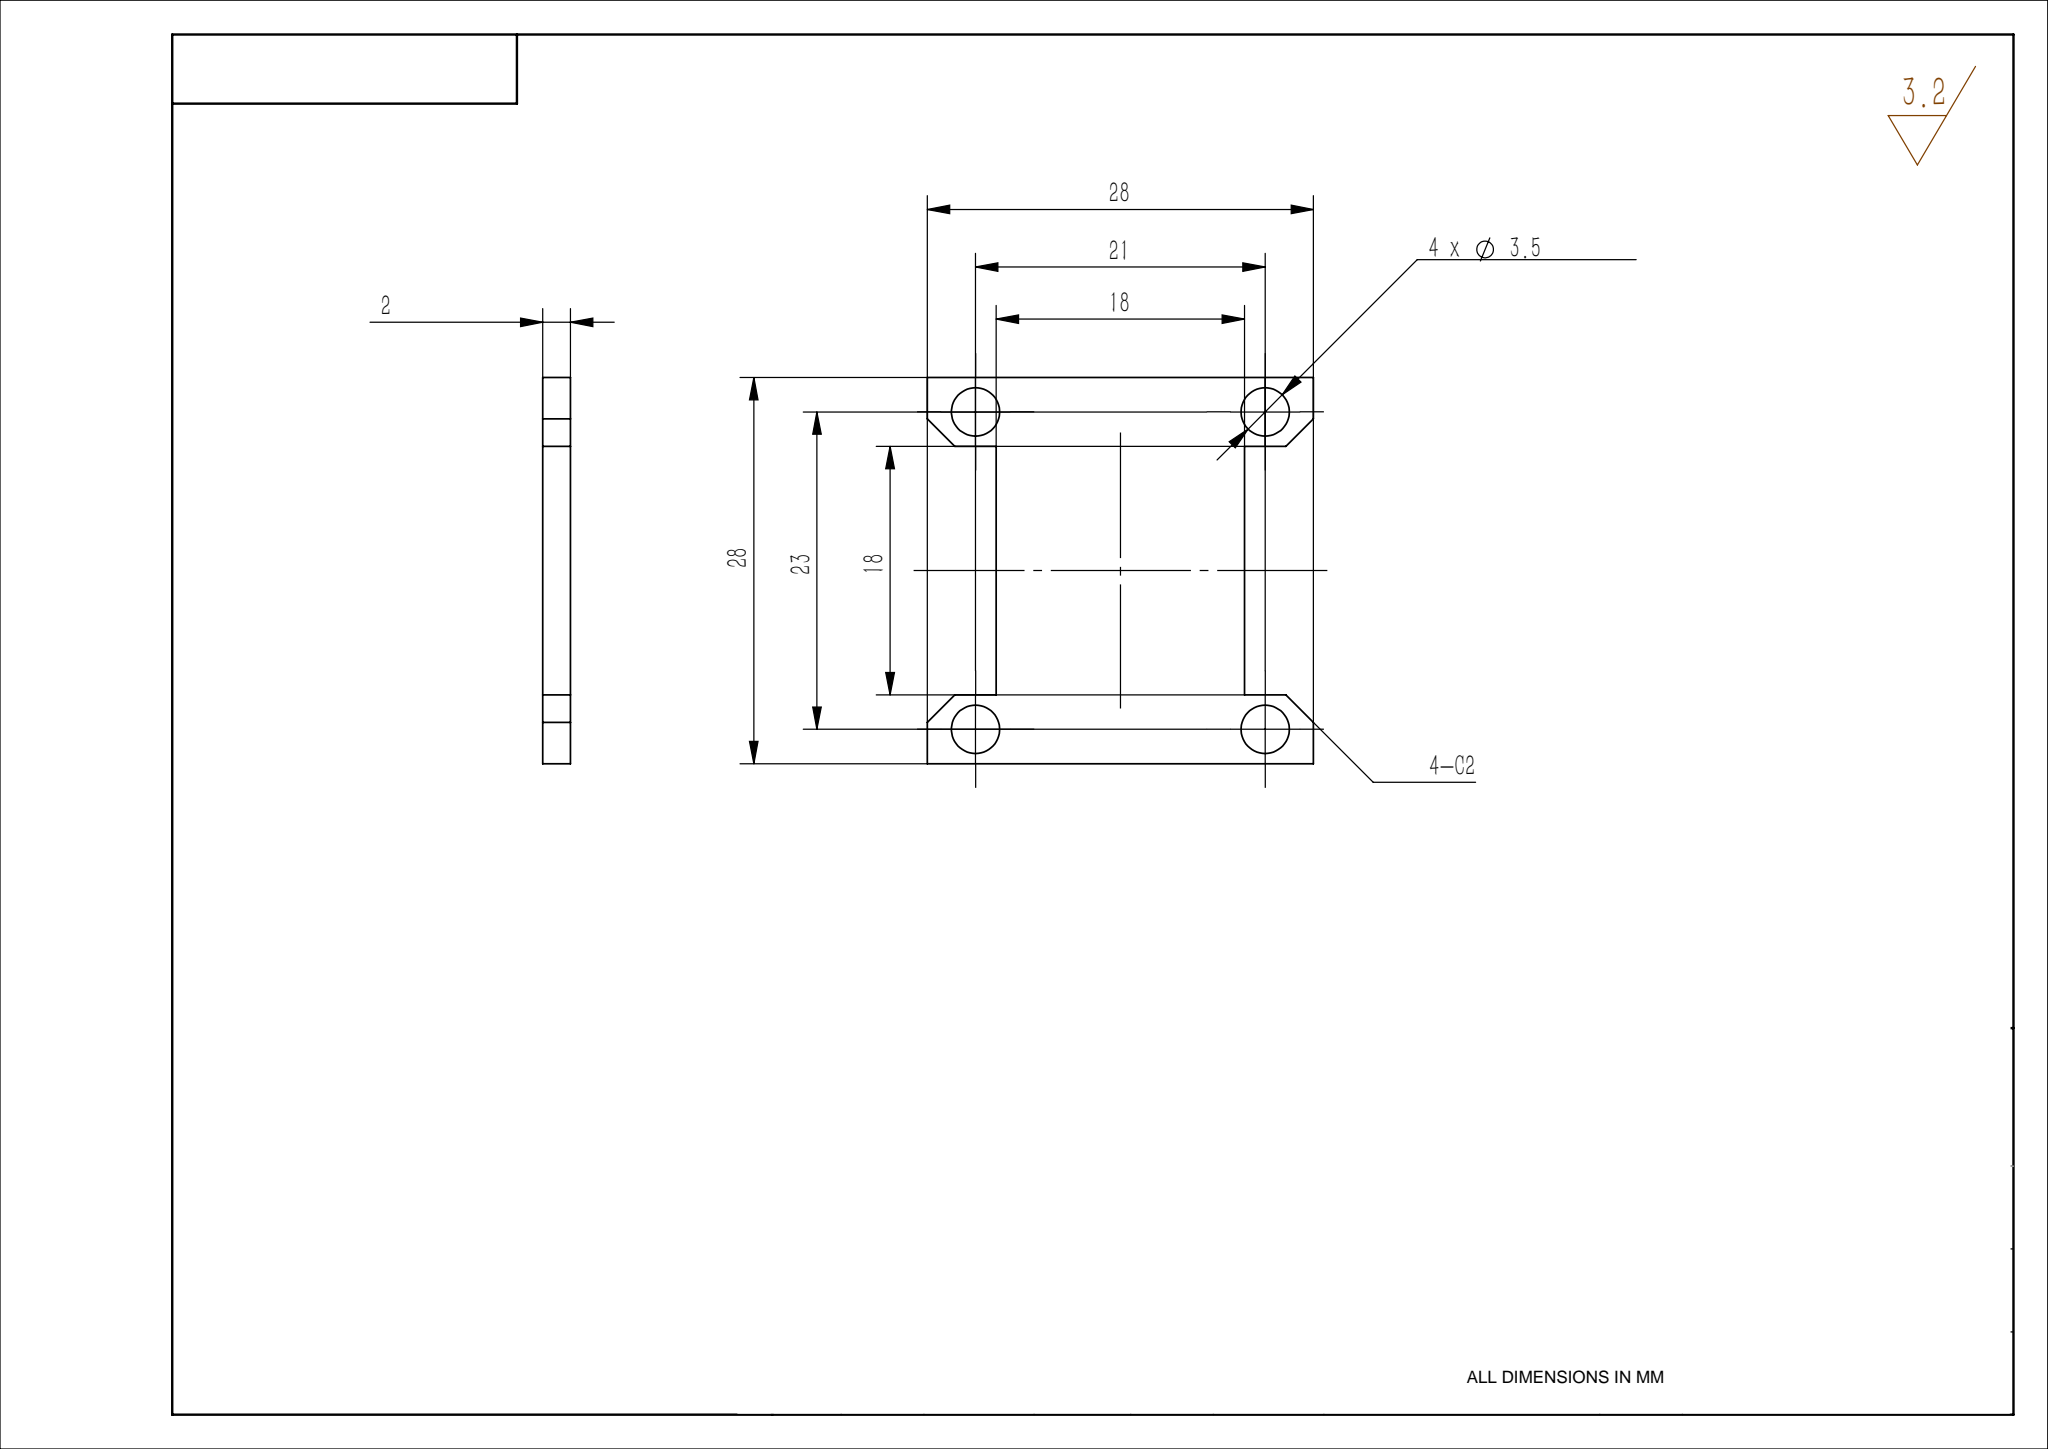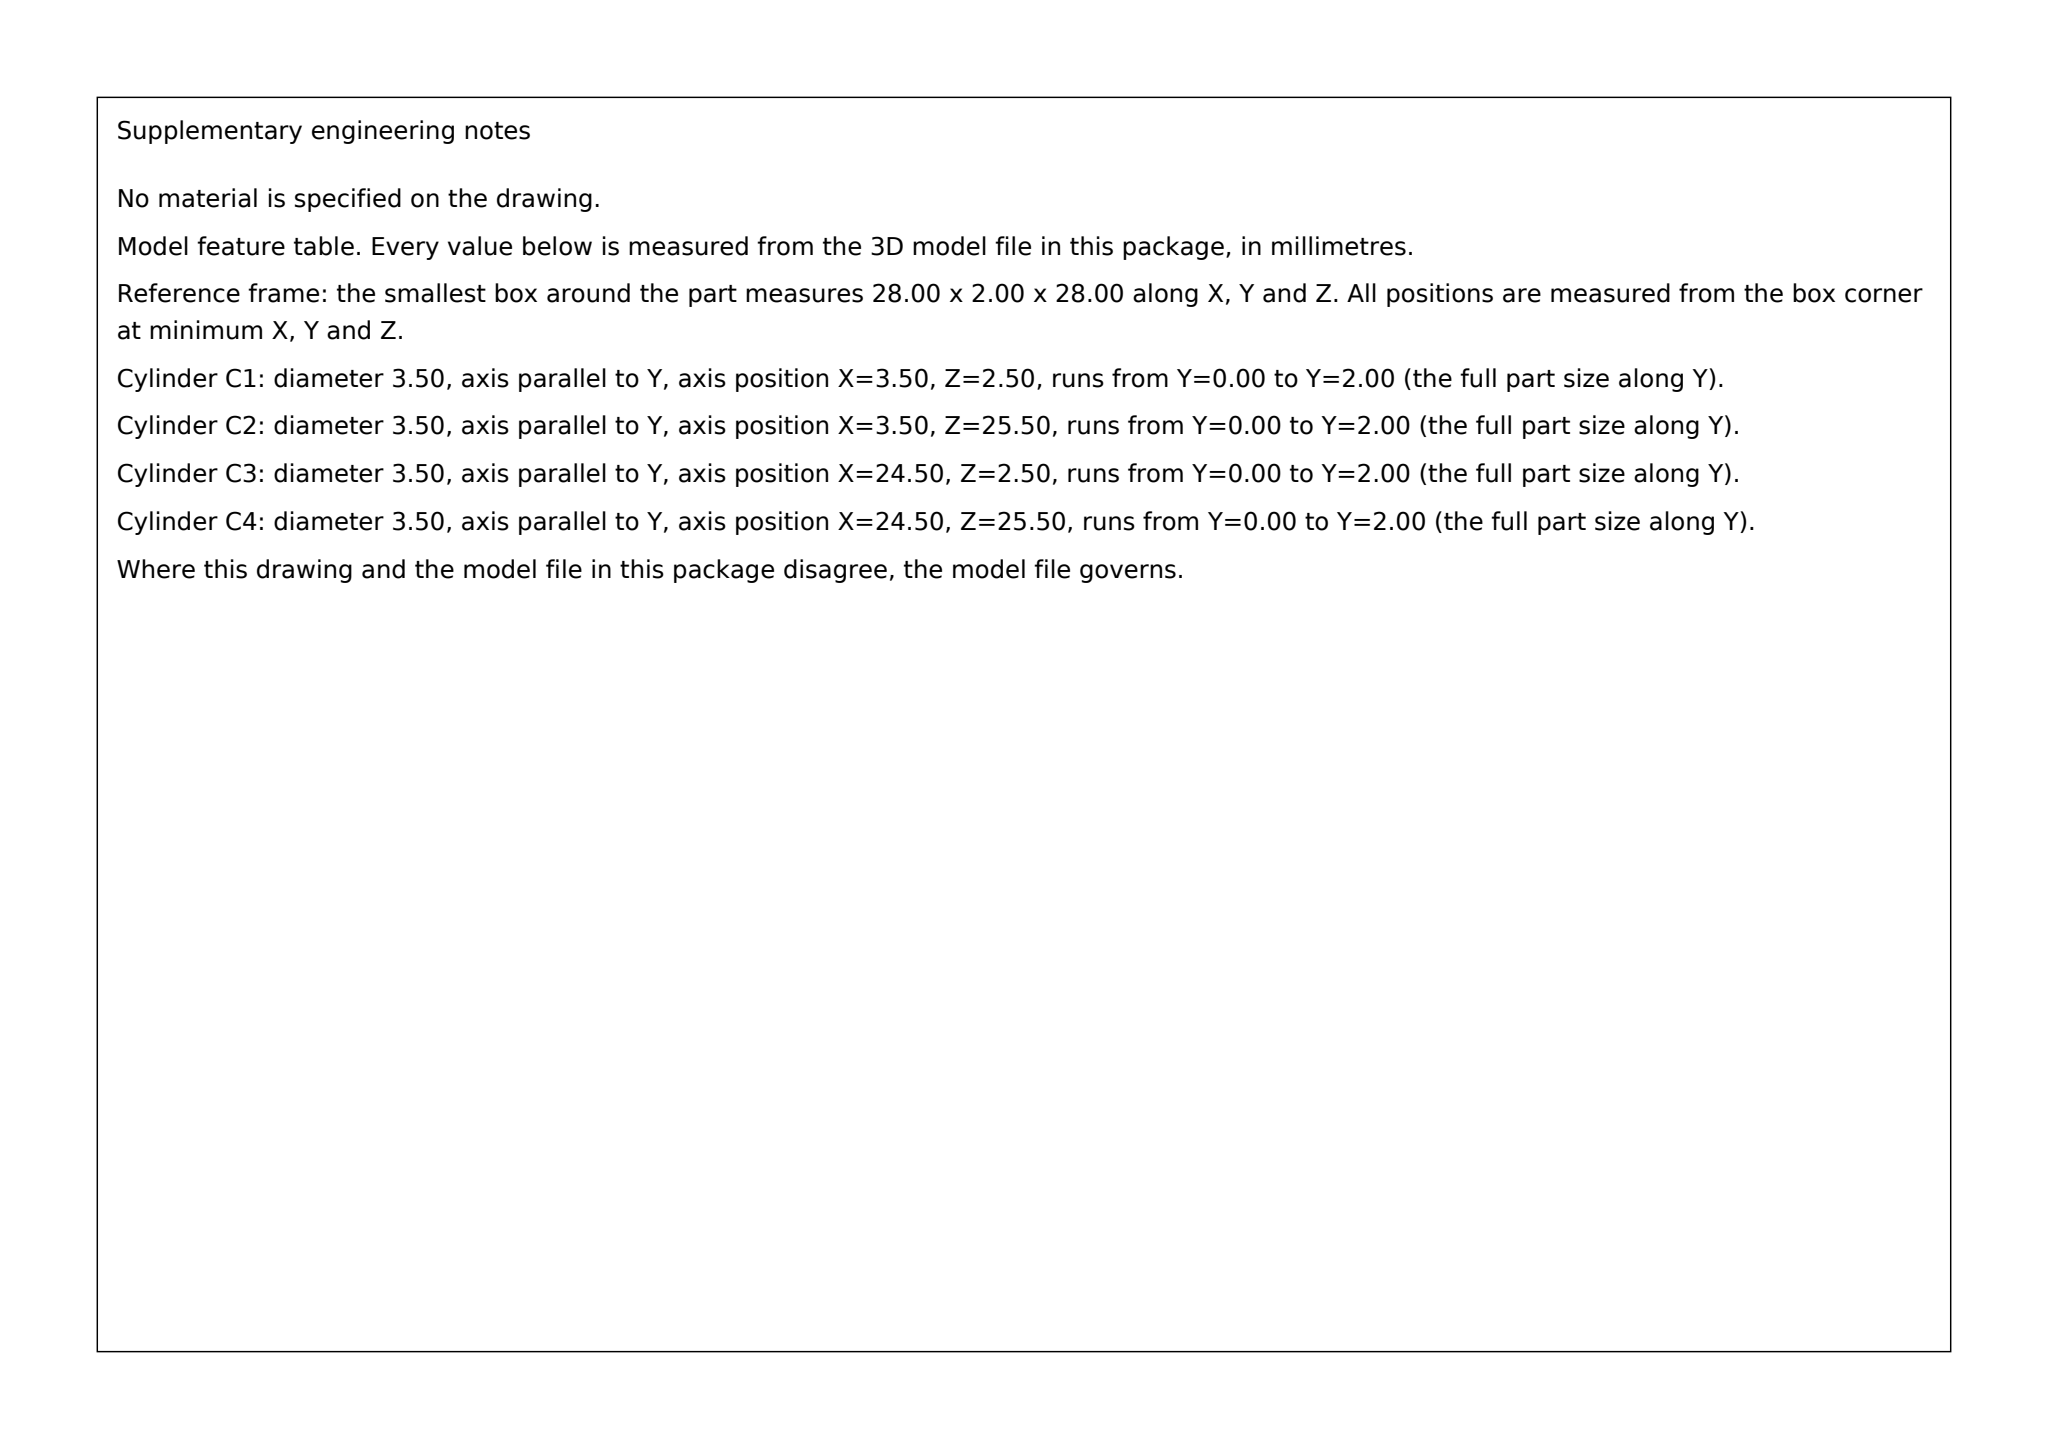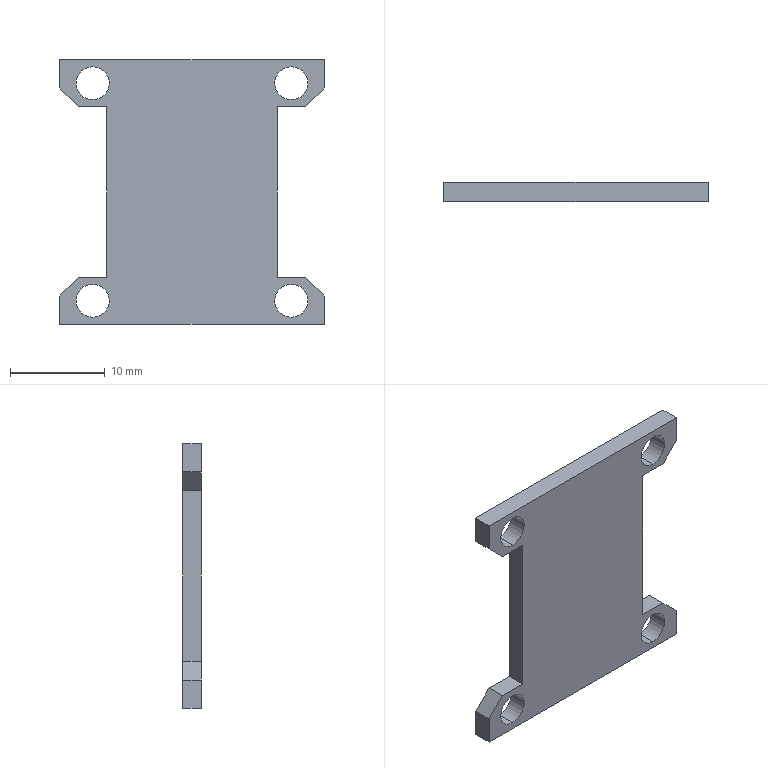Part | SolidWorks | mm | 1 solid | 26 faces | box 28 x 2 x 28 mm | volume 1115 mm3 | plane 18 | cylinder 8 | commonest cylinder face diameters 3.5 x8
STEP:
#1=CARTESIAN_POINT('',(-10.5,-2.,-13.25));
#2=VERTEX_POINT('',#1);
#3=CARTESIAN_POINT('',(-10.5,-2.,-9.75));
#4=VERTEX_POINT('',#3);
#5=CARTESIAN_POINT('',(-10.5,-2.,-11.5));
#6=DIRECTION('',(0.,1.,0.));
#7=DIRECTION('',(0.,0.,1.));
#8=AXIS2_PLACEMENT_3D('',#5,#6,#7);
#9=CIRCLE('',#8,1.75);
#10=EDGE_CURVE('',#2,#4,#9,.T.);
#11=ORIENTED_EDGE('',*,*,#10,.F.);
#12=CARTESIAN_POINT('',(-10.5,0.,-13.25));
#13=VERTEX_POINT('',#12);
#14=CARTESIAN_POINT('',(-10.5,0.,-13.25));
#15=DIRECTION('',(0.,1.,0.));
#16=VECTOR('',#15,1000.);
#17=LINE('',#14,#16);
#18=EDGE_CURVE('',#2,#13,#17,.T.);
#19=ORIENTED_EDGE('',*,*,#18,.T.);
#20=CARTESIAN_POINT('',(-10.5,0.,-9.75));
#21=VERTEX_POINT('',#20);
#22=CARTESIAN_POINT('',(-10.5,0.,-11.5));
#23=DIRECTION('',(0.,1.,0.));
#24=DIRECTION('',(0.,0.,1.));
#25=AXIS2_PLACEMENT_3D('',#22,#23,#24);
#26=CIRCLE('',#25,1.75);
#27=EDGE_CURVE('',#13,#21,#26,.T.);
#28=ORIENTED_EDGE('',*,*,#27,.T.);
#29=CARTESIAN_POINT('',(-10.5,0.,-9.75));
#30=DIRECTION('',(0.,1.,0.));
#31=VECTOR('',#30,1000.);
#32=LINE('',#29,#31);
#33=EDGE_CURVE('',#4,#21,#32,.T.);
#34=ORIENTED_EDGE('',*,*,#33,.F.);
#35=EDGE_LOOP('',(#11,#19,#28,#34));
#36=FACE_OUTER_BOUND('',#35,.T.);
#37=CARTESIAN_POINT('',(-10.5,0.,-11.5));
#38=DIRECTION('',(0.,1.,0.));
#39=DIRECTION('',(0.,0.,1.));
#40=AXIS2_PLACEMENT_3D('',#37,#38,#39);
#41=CYLINDRICAL_SURFACE('',#40,1.75);
#42=ADVANCED_FACE('',(#36),#41,.F.);
#43=CARTESIAN_POINT('',(10.5,-2.,-13.25));
#44=VERTEX_POINT('',#43);
#45=CARTESIAN_POINT('',(10.5,-2.,-9.75));
#46=VERTEX_POINT('',#45);
#47=CARTESIAN_POINT('',(10.5,-2.,-11.5));
#48=DIRECTION('',(0.,1.,0.));
#49=DIRECTION('',(0.,0.,1.));
#50=AXIS2_PLACEMENT_3D('',#47,#48,#49);
#51=CIRCLE('',#50,1.75);
#52=EDGE_CURVE('',#44,#46,#51,.T.);
#53=ORIENTED_EDGE('',*,*,#52,.F.);
#54=CARTESIAN_POINT('',(10.5,0.,-13.25));
#55=VERTEX_POINT('',#54);
#56=CARTESIAN_POINT('',(10.5,0.,-13.25));
#57=DIRECTION('',(0.,1.,0.));
#58=VECTOR('',#57,1000.);
#59=LINE('',#56,#58);
#60=EDGE_CURVE('',#44,#55,#59,.T.);
#61=ORIENTED_EDGE('',*,*,#60,.T.);
#62=CARTESIAN_POINT('',(10.5,0.,-9.75));
#63=VERTEX_POINT('',#62);
#64=CARTESIAN_POINT('',(10.5,0.,-11.5));
#65=DIRECTION('',(0.,1.,0.));
#66=DIRECTION('',(0.,0.,1.));
#67=AXIS2_PLACEMENT_3D('',#64,#65,#66);
#68=CIRCLE('',#67,1.75);
#69=EDGE_CURVE('',#55,#63,#68,.T.);
#70=ORIENTED_EDGE('',*,*,#69,.T.);
#71=CARTESIAN_POINT('',(10.5,0.,-9.75));
#72=DIRECTION('',(0.,1.,0.));
#73=VECTOR('',#72,1000.);
#74=LINE('',#71,#73);
#75=EDGE_CURVE('',#46,#63,#74,.T.);
#76=ORIENTED_EDGE('',*,*,#75,.F.);
#77=EDGE_LOOP('',(#53,#61,#70,#76));
#78=FACE_OUTER_BOUND('',#77,.T.);
#79=CARTESIAN_POINT('',(10.5,0.,-11.5));
#80=DIRECTION('',(0.,1.,0.));
#81=DIRECTION('',(0.,0.,1.));
#82=AXIS2_PLACEMENT_3D('',#79,#80,#81);
#83=CYLINDRICAL_SURFACE('',#82,1.75);
#84=ADVANCED_FACE('',(#78),#83,.F.);
#85=CARTESIAN_POINT('',(10.5,-2.,9.75));
#86=VERTEX_POINT('',#85);
#87=CARTESIAN_POINT('',(10.5,-2.,13.25));
#88=VERTEX_POINT('',#87);
#89=CARTESIAN_POINT('',(10.5,-2.,11.5));
#90=DIRECTION('',(0.,1.,0.));
#91=DIRECTION('',(0.,0.,1.));
#92=AXIS2_PLACEMENT_3D('',#89,#90,#91);
#93=CIRCLE('',#92,1.75);
#94=EDGE_CURVE('',#86,#88,#93,.T.);
#95=ORIENTED_EDGE('',*,*,#94,.F.);
#96=CARTESIAN_POINT('',(10.5,0.,9.75));
#97=VERTEX_POINT('',#96);
#98=CARTESIAN_POINT('',(10.5,0.,9.75));
#99=DIRECTION('',(0.,1.,0.));
#100=VECTOR('',#99,1000.);
#101=LINE('',#98,#100);
#102=EDGE_CURVE('',#86,#97,#101,.T.);
#103=ORIENTED_EDGE('',*,*,#102,.T.);
#104=CARTESIAN_POINT('',(10.5,0.,13.25));
#105=VERTEX_POINT('',#104);
#106=CARTESIAN_POINT('',(10.5,0.,11.5));
#107=DIRECTION('',(0.,1.,0.));
#108=DIRECTION('',(0.,0.,1.));
#109=AXIS2_PLACEMENT_3D('',#106,#107,#108);
#110=CIRCLE('',#109,1.75);
#111=EDGE_CURVE('',#97,#105,#110,.T.);
#112=ORIENTED_EDGE('',*,*,#111,.T.);
#113=CARTESIAN_POINT('',(10.5,0.,13.25));
#114=DIRECTION('',(0.,1.,0.));
#115=VECTOR('',#114,1000.);
#116=LINE('',#113,#115);
#117=EDGE_CURVE('',#88,#105,#116,.T.);
#118=ORIENTED_EDGE('',*,*,#117,.F.);
#119=EDGE_LOOP('',(#95,#103,#112,#118));
#120=FACE_OUTER_BOUND('',#119,.T.);
#121=CARTESIAN_POINT('',(10.5,0.,11.5));
#122=DIRECTION('',(0.,1.,0.));
#123=DIRECTION('',(0.,0.,1.));
#124=AXIS2_PLACEMENT_3D('',#121,#122,#123);
#125=CYLINDRICAL_SURFACE('',#124,1.75);
#126=ADVANCED_FACE('',(#120),#125,.F.);
#127=CARTESIAN_POINT('',(-10.5,-2.,9.75));
#128=VERTEX_POINT('',#127);
#129=CARTESIAN_POINT('',(-10.5,-2.,13.25));
#130=VERTEX_POINT('',#129);
#131=CARTESIAN_POINT('',(-10.5,-2.,11.5));
#132=DIRECTION('',(0.,1.,0.));
#133=DIRECTION('',(0.,0.,1.));
#134=AXIS2_PLACEMENT_3D('',#131,#132,#133);
#135=CIRCLE('',#134,1.75);
#136=EDGE_CURVE('',#128,#130,#135,.T.);
#137=ORIENTED_EDGE('',*,*,#136,.F.);
#138=CARTESIAN_POINT('',(-10.5,0.,9.75));
#139=VERTEX_POINT('',#138);
#140=CARTESIAN_POINT('',(-10.5,0.,9.75));
#141=DIRECTION('',(0.,1.,0.));
#142=VECTOR('',#141,1000.);
#143=LINE('',#140,#142);
#144=EDGE_CURVE('',#128,#139,#143,.T.);
#145=ORIENTED_EDGE('',*,*,#144,.T.);
#146=CARTESIAN_POINT('',(-10.5,0.,13.25));
#147=VERTEX_POINT('',#146);
#148=CARTESIAN_POINT('',(-10.5,0.,11.5));
#149=DIRECTION('',(0.,1.,0.));
#150=DIRECTION('',(0.,0.,1.));
#151=AXIS2_PLACEMENT_3D('',#148,#149,#150);
#152=CIRCLE('',#151,1.75);
#153=EDGE_CURVE('',#139,#147,#152,.T.);
#154=ORIENTED_EDGE('',*,*,#153,.T.);
#155=CARTESIAN_POINT('',(-10.5,0.,13.25));
#156=DIRECTION('',(0.,1.,0.));
#157=VECTOR('',#156,1000.);
#158=LINE('',#155,#157);
#159=EDGE_CURVE('',#130,#147,#158,.T.);
#160=ORIENTED_EDGE('',*,*,#159,.F.);
#161=EDGE_LOOP('',(#137,#145,#154,#160));
#162=FACE_OUTER_BOUND('',#161,.T.);
#163=CARTESIAN_POINT('',(-10.5,0.,11.5));
#164=DIRECTION('',(0.,1.,0.));
#165=DIRECTION('',(0.,0.,1.));
#166=AXIS2_PLACEMENT_3D('',#163,#164,#165);
#167=CYLINDRICAL_SURFACE('',#166,1.75);
#168=ADVANCED_FACE('',(#162),#167,.F.);
#169=CARTESIAN_POINT('',(14.,0.,-11.));
#170=VERTEX_POINT('',#169);
#171=CARTESIAN_POINT('',(14.,0.,-14.));
#172=VERTEX_POINT('',#171);
#173=CARTESIAN_POINT('',(14.,0.,14.));
#174=DIRECTION('',(0.,0.,-1.));
#175=VECTOR('',#174,1000.);
#176=LINE('',#173,#175);
#177=EDGE_CURVE('',#170,#172,#176,.T.);
#178=ORIENTED_EDGE('',*,*,#177,.F.);
#179=CARTESIAN_POINT('',(14.,-2.,-11.));
#180=VERTEX_POINT('',#179);
#181=CARTESIAN_POINT('',(14.,-2.,-11.));
#182=DIRECTION('',(0.,-1.,0.));
#183=VECTOR('',#182,1000.);
#184=LINE('',#181,#183);
#185=EDGE_CURVE('',#170,#180,#184,.T.);
#186=ORIENTED_EDGE('',*,*,#185,.T.);
#187=CARTESIAN_POINT('',(14.,-2.,-14.));
#188=VERTEX_POINT('',#187);
#189=CARTESIAN_POINT('',(14.,-2.,14.));
#190=DIRECTION('',(0.,0.,-1.));
#191=VECTOR('',#190,1000.);
#192=LINE('',#189,#191);
#193=EDGE_CURVE('',#180,#188,#192,.T.);
#194=ORIENTED_EDGE('',*,*,#193,.T.);
#195=CARTESIAN_POINT('',(14.,-2.,-14.));
#196=DIRECTION('',(0.,1.,0.));
#197=VECTOR('',#196,1000.);
#198=LINE('',#195,#197);
#199=EDGE_CURVE('',#188,#172,#198,.T.);
#200=ORIENTED_EDGE('',*,*,#199,.T.);
#201=EDGE_LOOP('',(#178,#186,#194,#200));
#202=FACE_OUTER_BOUND('',#201,.T.);
#203=CARTESIAN_POINT('',(14.,-2.,14.));
#204=DIRECTION('',(1.,0.,0.));
#205=DIRECTION('',(0.,0.,-1.));
#206=AXIS2_PLACEMENT_3D('',#203,#204,#205);
#207=PLANE('',#206);
#208=ADVANCED_FACE('',(#202),#207,.T.);
#209=CARTESIAN_POINT('',(-14.,-2.,-14.));
#210=VERTEX_POINT('',#209);
#211=CARTESIAN_POINT('',(-14.,-2.,-11.));
#212=VERTEX_POINT('',#211);
#213=CARTESIAN_POINT('',(-14.,-2.,14.));
#214=DIRECTION('',(0.,0.,1.));
#215=VECTOR('',#214,1000.);
#216=LINE('',#213,#215);
#217=EDGE_CURVE('',#210,#212,#216,.T.);
#218=ORIENTED_EDGE('',*,*,#217,.T.);
#219=CARTESIAN_POINT('',(-14.,0.,-11.));
#220=VERTEX_POINT('',#219);
#221=CARTESIAN_POINT('',(-14.,0.,-11.));
#222=DIRECTION('',(0.,1.,0.));
#223=VECTOR('',#222,1000.);
#224=LINE('',#221,#223);
#225=EDGE_CURVE('',#212,#220,#224,.T.);
#226=ORIENTED_EDGE('',*,*,#225,.T.);
#227=CARTESIAN_POINT('',(-14.,0.,-14.));
#228=VERTEX_POINT('',#227);
#229=CARTESIAN_POINT('',(-14.,0.,14.));
#230=DIRECTION('',(0.,0.,1.));
#231=VECTOR('',#230,1000.);
#232=LINE('',#229,#231);
#233=EDGE_CURVE('',#228,#220,#232,.T.);
#234=ORIENTED_EDGE('',*,*,#233,.F.);
#235=CARTESIAN_POINT('',(-14.,-2.,-14.));
#236=DIRECTION('',(0.,1.,0.));
#237=VECTOR('',#236,1000.);
#238=LINE('',#235,#237);
#239=EDGE_CURVE('',#210,#228,#238,.T.);
#240=ORIENTED_EDGE('',*,*,#239,.F.);
#241=EDGE_LOOP('',(#218,#226,#234,#240));
#242=FACE_OUTER_BOUND('',#241,.T.);
#243=CARTESIAN_POINT('',(-14.,-2.,14.));
#244=DIRECTION('',(-1.,0.,0.));
#245=DIRECTION('',(0.,0.,1.));
#246=AXIS2_PLACEMENT_3D('',#243,#244,#245);
#247=PLANE('',#246);
#248=ADVANCED_FACE('',(#242),#247,.T.);
#249=CARTESIAN_POINT('',(14.,-2.,14.));
#250=VERTEX_POINT('',#249);
#251=CARTESIAN_POINT('',(14.,-2.,11.));
#252=VERTEX_POINT('',#251);
#253=CARTESIAN_POINT('',(14.,-2.,14.));
#254=DIRECTION('',(0.,0.,-1.));
#255=VECTOR('',#254,1000.);
#256=LINE('',#253,#255);
#257=EDGE_CURVE('',#250,#252,#256,.T.);
#258=ORIENTED_EDGE('',*,*,#257,.T.);
#259=CARTESIAN_POINT('',(14.,0.,11.));
#260=VERTEX_POINT('',#259);
#261=CARTESIAN_POINT('',(14.,0.,11.));
#262=DIRECTION('',(0.,1.,0.));
#263=VECTOR('',#262,1000.);
#264=LINE('',#261,#263);
#265=EDGE_CURVE('',#252,#260,#264,.T.);
#266=ORIENTED_EDGE('',*,*,#265,.T.);
#267=CARTESIAN_POINT('',(14.,0.,14.));
#268=VERTEX_POINT('',#267);
#269=CARTESIAN_POINT('',(14.,0.,14.));
#270=DIRECTION('',(0.,0.,-1.));
#271=VECTOR('',#270,1000.);
#272=LINE('',#269,#271);
#273=EDGE_CURVE('',#268,#260,#272,.T.);
#274=ORIENTED_EDGE('',*,*,#273,.F.);
#275=CARTESIAN_POINT('',(14.,-2.,14.));
#276=DIRECTION('',(0.,1.,0.));
#277=VECTOR('',#276,1000.);
#278=LINE('',#275,#277);
#279=EDGE_CURVE('',#250,#268,#278,.T.);
#280=ORIENTED_EDGE('',*,*,#279,.F.);
#281=EDGE_LOOP('',(#258,#266,#274,#280));
#282=FACE_OUTER_BOUND('',#281,.T.);
#283=CARTESIAN_POINT('',(14.,-2.,14.));
#284=DIRECTION('',(1.,0.,0.));
#285=DIRECTION('',(0.,0.,-1.));
#286=AXIS2_PLACEMENT_3D('',#283,#284,#285);
#287=PLANE('',#286);
#288=ADVANCED_FACE('',(#282),#287,.T.);
#289=CARTESIAN_POINT('',(-14.,0.,14.));
#290=VERTEX_POINT('',#289);
#291=CARTESIAN_POINT('',(-14.,0.,14.));
#292=DIRECTION('',(1.,0.,0.));
#293=VECTOR('',#292,1000.);
#294=LINE('',#291,#293);
#295=EDGE_CURVE('',#290,#268,#294,.T.);
#296=ORIENTED_EDGE('',*,*,#295,.F.);
#297=CARTESIAN_POINT('',(-14.,-2.,14.));
#298=VERTEX_POINT('',#297);
#299=CARTESIAN_POINT('',(-14.,-2.,14.));
#300=DIRECTION('',(0.,1.,0.));
#301=VECTOR('',#300,1000.);
#302=LINE('',#299,#301);
#303=EDGE_CURVE('',#298,#290,#302,.T.);
#304=ORIENTED_EDGE('',*,*,#303,.F.);
#305=CARTESIAN_POINT('',(-14.,-2.,14.));
#306=DIRECTION('',(1.,0.,0.));
#307=VECTOR('',#306,1000.);
#308=LINE('',#305,#307);
#309=EDGE_CURVE('',#298,#250,#308,.T.);
#310=ORIENTED_EDGE('',*,*,#309,.T.);
#311=ORIENTED_EDGE('',*,*,#279,.T.);
#312=EDGE_LOOP('',(#296,#304,#310,#311));
#313=FACE_OUTER_BOUND('',#312,.T.);
#314=CARTESIAN_POINT('',(-14.,-2.,14.));
#315=DIRECTION('',(0.,0.,1.));
#316=DIRECTION('',(1.,0.,0.));
#317=AXIS2_PLACEMENT_3D('',#314,#315,#316);
#318=PLANE('',#317);
#319=ADVANCED_FACE('',(#313),#318,.T.);
#320=CARTESIAN_POINT('',(-14.,0.,11.));
#321=VERTEX_POINT('',#320);
#322=CARTESIAN_POINT('',(-14.,0.,14.));
#323=DIRECTION('',(0.,0.,1.));
#324=VECTOR('',#323,1000.);
#325=LINE('',#322,#324);
#326=EDGE_CURVE('',#321,#290,#325,.T.);
#327=ORIENTED_EDGE('',*,*,#326,.F.);
#328=CARTESIAN_POINT('',(-14.,-2.,11.));
#329=VERTEX_POINT('',#328);
#330=CARTESIAN_POINT('',(-14.,-2.,11.));
#331=DIRECTION('',(0.,-1.,0.));
#332=VECTOR('',#331,1000.);
#333=LINE('',#330,#332);
#334=EDGE_CURVE('',#321,#329,#333,.T.);
#335=ORIENTED_EDGE('',*,*,#334,.T.);
#336=CARTESIAN_POINT('',(-14.,-2.,14.));
#337=DIRECTION('',(0.,0.,1.));
#338=VECTOR('',#337,1000.);
#339=LINE('',#336,#338);
#340=EDGE_CURVE('',#329,#298,#339,.T.);
#341=ORIENTED_EDGE('',*,*,#340,.T.);
#342=ORIENTED_EDGE('',*,*,#303,.T.);
#343=EDGE_LOOP('',(#327,#335,#341,#342));
#344=FACE_OUTER_BOUND('',#343,.T.);
#345=CARTESIAN_POINT('',(-14.,-2.,14.));
#346=DIRECTION('',(-1.,0.,0.));
#347=DIRECTION('',(0.,0.,1.));
#348=AXIS2_PLACEMENT_3D('',#345,#346,#347);
#349=PLANE('',#348);
#350=ADVANCED_FACE('',(#344),#349,.T.);
#351=CARTESIAN_POINT('',(-14.,0.,-14.));
#352=DIRECTION('',(-1.,0.,0.));
#353=VECTOR('',#352,1000.);
#354=LINE('',#351,#353);
#355=EDGE_CURVE('',#172,#228,#354,.T.);
#356=ORIENTED_EDGE('',*,*,#355,.F.);
#357=ORIENTED_EDGE('',*,*,#199,.F.);
#358=CARTESIAN_POINT('',(-14.,-2.,-14.));
#359=DIRECTION('',(-1.,0.,0.));
#360=VECTOR('',#359,1000.);
#361=LINE('',#358,#360);
#362=EDGE_CURVE('',#188,#210,#361,.T.);
#363=ORIENTED_EDGE('',*,*,#362,.T.);
#364=ORIENTED_EDGE('',*,*,#239,.T.);
#365=EDGE_LOOP('',(#356,#357,#363,#364));
#366=FACE_OUTER_BOUND('',#365,.T.);
#367=CARTESIAN_POINT('',(-14.,-2.,-14.));
#368=DIRECTION('',(0.,0.,-1.));
#369=DIRECTION('',(-1.,0.,0.));
#370=AXIS2_PLACEMENT_3D('',#367,#368,#369);
#371=PLANE('',#370);
#372=ADVANCED_FACE('',(#366),#371,.T.);
#373=CARTESIAN_POINT('',(-10.5,-2.,-11.5));
#374=DIRECTION('',(0.,1.,0.));
#375=DIRECTION('',(0.,0.,1.));
#376=AXIS2_PLACEMENT_3D('',#373,#374,#375);
#377=CIRCLE('',#376,1.75);
#378=EDGE_CURVE('',#4,#2,#377,.T.);
#379=ORIENTED_EDGE('',*,*,#378,.T.);
#380=ORIENTED_EDGE('',*,*,#10,.T.);
#381=EDGE_LOOP('',(#379,#380));
#382=FACE_BOUND('',#381,.T.);
#383=CARTESIAN_POINT('',(10.5,-2.,-11.5));
#384=DIRECTION('',(0.,1.,0.));
#385=DIRECTION('',(0.,0.,1.));
#386=AXIS2_PLACEMENT_3D('',#383,#384,#385);
#387=CIRCLE('',#386,1.75);
#388=EDGE_CURVE('',#46,#44,#387,.T.);
#389=ORIENTED_EDGE('',*,*,#388,.T.);
#390=ORIENTED_EDGE('',*,*,#52,.T.);
#391=EDGE_LOOP('',(#389,#390));
#392=FACE_BOUND('',#391,.T.);
#393=CARTESIAN_POINT('',(10.5,-2.,11.5));
#394=DIRECTION('',(0.,1.,0.));
#395=DIRECTION('',(0.,0.,1.));
#396=AXIS2_PLACEMENT_3D('',#393,#394,#395);
#397=CIRCLE('',#396,1.75);
#398=EDGE_CURVE('',#88,#86,#397,.T.);
#399=ORIENTED_EDGE('',*,*,#398,.T.);
#400=ORIENTED_EDGE('',*,*,#94,.T.);
#401=EDGE_LOOP('',(#399,#400));
#402=FACE_BOUND('',#401,.T.);
#403=CARTESIAN_POINT('',(-10.5,-2.,11.5));
#404=DIRECTION('',(0.,1.,0.));
#405=DIRECTION('',(0.,0.,1.));
#406=AXIS2_PLACEMENT_3D('',#403,#404,#405);
#407=CIRCLE('',#406,1.75);
#408=EDGE_CURVE('',#130,#128,#407,.T.);
#409=ORIENTED_EDGE('',*,*,#408,.T.);
#410=ORIENTED_EDGE('',*,*,#136,.T.);
#411=EDGE_LOOP('',(#409,#410));
#412=FACE_BOUND('',#411,.T.);
#413=CARTESIAN_POINT('',(12.,-2.,9.));
#414=VERTEX_POINT('',#413);
#415=CARTESIAN_POINT('',(9.,-2.,9.));
#416=VERTEX_POINT('',#415);
#417=CARTESIAN_POINT('',(0.,-2.,9.));
#418=DIRECTION('',(-1.,0.,0.));
#419=VECTOR('',#418,1000.);
#420=LINE('',#417,#419);
#421=EDGE_CURVE('',#414,#416,#420,.T.);
#422=ORIENTED_EDGE('',*,*,#421,.F.);
#423=CARTESIAN_POINT('',(1.5,-2.,-1.5));
#424=DIRECTION('',(0.7071,0.,0.7071));
#425=VECTOR('',#424,1000.);
#426=LINE('',#423,#425);
#427=EDGE_CURVE('',#414,#252,#426,.T.);
#428=ORIENTED_EDGE('',*,*,#427,.T.);
#429=ORIENTED_EDGE('',*,*,#257,.F.);
#430=ORIENTED_EDGE('',*,*,#309,.F.);
#431=ORIENTED_EDGE('',*,*,#340,.F.);
#432=CARTESIAN_POINT('',(-12.,-2.,9.));
#433=VERTEX_POINT('',#432);
#434=CARTESIAN_POINT('',(-1.5,-2.,-1.5));
#435=DIRECTION('',(0.7071,0.,-0.7071));
#436=VECTOR('',#435,1000.);
#437=LINE('',#434,#436);
#438=EDGE_CURVE('',#329,#433,#437,.T.);
#439=ORIENTED_EDGE('',*,*,#438,.T.);
#440=CARTESIAN_POINT('',(-9.,-2.,9.));
#441=VERTEX_POINT('',#440);
#442=CARTESIAN_POINT('',(0.,-2.,9.));
#443=DIRECTION('',(-1.,0.,0.));
#444=VECTOR('',#443,1000.);
#445=LINE('',#442,#444);
#446=EDGE_CURVE('',#441,#433,#445,.T.);
#447=ORIENTED_EDGE('',*,*,#446,.F.);
#448=CARTESIAN_POINT('',(-9.,-2.,-9.));
#449=VERTEX_POINT('',#448);
#450=CARTESIAN_POINT('',(-9.,-2.,0.));
#451=DIRECTION('',(0.,0.,1.));
#452=VECTOR('',#451,1000.);
#453=LINE('',#450,#452);
#454=EDGE_CURVE('',#449,#441,#453,.T.);
#455=ORIENTED_EDGE('',*,*,#454,.F.);
#456=CARTESIAN_POINT('',(-12.,-2.,-9.));
#457=VERTEX_POINT('',#456);
#458=CARTESIAN_POINT('',(0.,-2.,-9.));
#459=DIRECTION('',(1.,0.,0.));
#460=VECTOR('',#459,1000.);
#461=LINE('',#458,#460);
#462=EDGE_CURVE('',#457,#449,#461,.T.);
#463=ORIENTED_EDGE('',*,*,#462,.F.);
#464=CARTESIAN_POINT('',(-1.5,-2.,1.5));
#465=DIRECTION('',(-0.7071,0.,-0.7071));
#466=VECTOR('',#465,1000.);
#467=LINE('',#464,#466);
#468=EDGE_CURVE('',#457,#212,#467,.T.);
#469=ORIENTED_EDGE('',*,*,#468,.T.);
#470=ORIENTED_EDGE('',*,*,#217,.F.);
#471=ORIENTED_EDGE('',*,*,#362,.F.);
#472=ORIENTED_EDGE('',*,*,#193,.F.);
#473=CARTESIAN_POINT('',(12.,-2.,-9.));
#474=VERTEX_POINT('',#473);
#475=CARTESIAN_POINT('',(1.5,-2.,1.5));
#476=DIRECTION('',(-0.7071,0.,0.7071));
#477=VECTOR('',#476,1000.);
#478=LINE('',#475,#477);
#479=EDGE_CURVE('',#180,#474,#478,.T.);
#480=ORIENTED_EDGE('',*,*,#479,.T.);
#481=CARTESIAN_POINT('',(9.,-2.,-9.));
#482=VERTEX_POINT('',#481);
#483=CARTESIAN_POINT('',(-0.,-2.,-9.));
#484=DIRECTION('',(1.,0.,-0.));
#485=VECTOR('',#484,1000.);
#486=LINE('',#483,#485);
#487=EDGE_CURVE('',#482,#474,#486,.T.);
#488=ORIENTED_EDGE('',*,*,#487,.F.);
#489=CARTESIAN_POINT('',(9.,-2.,-0.));
#490=DIRECTION('',(-0.,0.,-1.));
#491=VECTOR('',#490,1000.);
#492=LINE('',#489,#491);
#493=EDGE_CURVE('',#416,#482,#492,.T.);
#494=ORIENTED_EDGE('',*,*,#493,.F.);
#495=EDGE_LOOP('',(#422,#428,#429,#430,#431,#439,#447,#455,#463,#469,#470,#471,#472,#480,#488,#494));
#496=FACE_OUTER_BOUND('',#495,.T.);
#497=CARTESIAN_POINT('',(0.,-2.,0.));
#498=DIRECTION('',(0.,-1.,0.));
#499=DIRECTION('',(0.,0.,-1.));
#500=AXIS2_PLACEMENT_3D('',#497,#498,#499);
#501=PLANE('',#500);
#502=ADVANCED_FACE('',(#382,#392,#402,#412,#496),#501,.T.);
#503=CARTESIAN_POINT('',(-10.5,0.,-11.5));
#504=DIRECTION('',(0.,1.,0.));
#505=DIRECTION('',(0.,0.,1.));
#506=AXIS2_PLACEMENT_3D('',#503,#504,#505);
#507=CIRCLE('',#506,1.75);
#508=EDGE_CURVE('',#21,#13,#507,.T.);
#509=ORIENTED_EDGE('',*,*,#508,.F.);
#510=ORIENTED_EDGE('',*,*,#27,.F.);
#511=EDGE_LOOP('',(#509,#510));
#512=FACE_BOUND('',#511,.T.);
#513=CARTESIAN_POINT('',(10.5,0.,-11.5));
#514=DIRECTION('',(0.,1.,0.));
#515=DIRECTION('',(0.,0.,1.));
#516=AXIS2_PLACEMENT_3D('',#513,#514,#515);
#517=CIRCLE('',#516,1.75);
#518=EDGE_CURVE('',#63,#55,#517,.T.);
#519=ORIENTED_EDGE('',*,*,#518,.F.);
#520=ORIENTED_EDGE('',*,*,#69,.F.);
#521=EDGE_LOOP('',(#519,#520));
#522=FACE_BOUND('',#521,.T.);
#523=CARTESIAN_POINT('',(10.5,0.,11.5));
#524=DIRECTION('',(0.,1.,0.));
#525=DIRECTION('',(0.,0.,1.));
#526=AXIS2_PLACEMENT_3D('',#523,#524,#525);
#527=CIRCLE('',#526,1.75);
#528=EDGE_CURVE('',#105,#97,#527,.T.);
#529=ORIENTED_EDGE('',*,*,#528,.F.);
#530=ORIENTED_EDGE('',*,*,#111,.F.);
#531=EDGE_LOOP('',(#529,#530));
#532=FACE_BOUND('',#531,.T.);
#533=CARTESIAN_POINT('',(-10.5,0.,11.5));
#534=DIRECTION('',(0.,1.,0.));
#535=DIRECTION('',(0.,0.,1.));
#536=AXIS2_PLACEMENT_3D('',#533,#534,#535);
#537=CIRCLE('',#536,1.75);
#538=EDGE_CURVE('',#147,#139,#537,.T.);
#539=ORIENTED_EDGE('',*,*,#538,.F.);
#540=ORIENTED_EDGE('',*,*,#153,.F.);
#541=EDGE_LOOP('',(#539,#540));
#542=FACE_BOUND('',#541,.T.);
#543=ORIENTED_EDGE('',*,*,#273,.T.);
#544=CARTESIAN_POINT('',(12.,0.,9.));
#545=VERTEX_POINT('',#544);
#546=CARTESIAN_POINT('',(12.,0.,9.));
#547=DIRECTION('',(-0.7071,0.,-0.7071));
#548=VECTOR('',#547,1000.);
#549=LINE('',#546,#548);
#550=EDGE_CURVE('',#260,#545,#549,.T.);
#551=ORIENTED_EDGE('',*,*,#550,.T.);
#552=CARTESIAN_POINT('',(9.,0.,9.));
#553=VERTEX_POINT('',#552);
#554=CARTESIAN_POINT('',(18.428,0.,9.));
#555=DIRECTION('',(1.,0.,-0.));
#556=VECTOR('',#555,1000.);
#557=LINE('',#554,#556);
#558=EDGE_CURVE('',#553,#545,#557,.T.);
#559=ORIENTED_EDGE('',*,*,#558,.F.);
#560=CARTESIAN_POINT('',(9.,0.,-9.));
#561=VERTEX_POINT('',#560);
#562=CARTESIAN_POINT('',(9.,0.,-9.));
#563=DIRECTION('',(0.,0.,1.));
#564=VECTOR('',#563,1000.);
#565=LINE('',#562,#564);
#566=EDGE_CURVE('',#561,#553,#565,.T.);
#567=ORIENTED_EDGE('',*,*,#566,.F.);
#568=CARTESIAN_POINT('',(12.,0.,-9.));
#569=VERTEX_POINT('',#568);
#570=CARTESIAN_POINT('',(-0.,0.,-9.));
#571=DIRECTION('',(1.,0.,-0.));
#572=VECTOR('',#571,1000.);
#573=LINE('',#570,#572);
#574=EDGE_CURVE('',#561,#569,#573,.T.);
#575=ORIENTED_EDGE('',*,*,#574,.T.);
#576=CARTESIAN_POINT('',(12.,0.,-9.));
#577=DIRECTION('',(0.7071,0.,-0.7071));
#578=VECTOR('',#577,1000.);
#579=LINE('',#576,#578);
#580=EDGE_CURVE('',#569,#170,#579,.T.);
#581=ORIENTED_EDGE('',*,*,#580,.T.);
#582=ORIENTED_EDGE('',*,*,#177,.T.);
#583=ORIENTED_EDGE('',*,*,#355,.T.);
#584=ORIENTED_EDGE('',*,*,#233,.T.);
#585=CARTESIAN_POINT('',(-12.,0.,-9.));
#586=VERTEX_POINT('',#585);
#587=CARTESIAN_POINT('',(-12.,0.,-9.));
#588=DIRECTION('',(0.7071,0.,0.7071));
#589=VECTOR('',#588,1000.);
#590=LINE('',#587,#589);
#591=EDGE_CURVE('',#220,#586,#590,.T.);
#592=ORIENTED_EDGE('',*,*,#591,.T.);
#593=CARTESIAN_POINT('',(-9.,0.,-9.));
#594=VERTEX_POINT('',#593);
#595=CARTESIAN_POINT('',(-18.428,0.,-9.));
#596=DIRECTION('',(-1.,0.,0.));
#597=VECTOR('',#596,1000.);
#598=LINE('',#595,#597);
#599=EDGE_CURVE('',#594,#586,#598,.T.);
#600=ORIENTED_EDGE('',*,*,#599,.F.);
#601=CARTESIAN_POINT('',(-9.,0.,9.));
#602=VERTEX_POINT('',#601);
#603=CARTESIAN_POINT('',(-9.,0.,-9.));
#604=DIRECTION('',(-0.,0.,-1.));
#605=VECTOR('',#604,1000.);
#606=LINE('',#603,#605);
#607=EDGE_CURVE('',#602,#594,#606,.T.);
#608=ORIENTED_EDGE('',*,*,#607,.F.);
#609=CARTESIAN_POINT('',(-12.,0.,9.));
#610=VERTEX_POINT('',#609);
#611=CARTESIAN_POINT('',(0.,0.,9.));
#612=DIRECTION('',(-1.,0.,0.));
#613=VECTOR('',#612,1000.);
#614=LINE('',#611,#613);
#615=EDGE_CURVE('',#602,#610,#614,.T.);
#616=ORIENTED_EDGE('',*,*,#615,.T.);
#617=CARTESIAN_POINT('',(-12.,0.,9.));
#618=DIRECTION('',(-0.7071,0.,0.7071));
#619=VECTOR('',#618,1000.);
#620=LINE('',#617,#619);
#621=EDGE_CURVE('',#610,#321,#620,.T.);
#622=ORIENTED_EDGE('',*,*,#621,.T.);
#623=ORIENTED_EDGE('',*,*,#326,.T.);
#624=ORIENTED_EDGE('',*,*,#295,.T.);
#625=EDGE_LOOP('',(#543,#551,#559,#567,#575,#581,#582,#583,#584,#592,#600,#608,#616,#622,#623,#624));
#626=FACE_OUTER_BOUND('',#625,.T.);
#627=CARTESIAN_POINT('',(0.,0.,0.));
#628=DIRECTION('',(0.,-1.,0.));
#629=DIRECTION('',(0.,0.,-1.));
#630=AXIS2_PLACEMENT_3D('',#627,#628,#629);
#631=PLANE('',#630);
#632=ADVANCED_FACE('',(#512,#522,#532,#542,#626),#631,.F.);
#633=ORIENTED_EDGE('',*,*,#599,.T.);
#634=CARTESIAN_POINT('',(-12.,-2.,-9.));
#635=DIRECTION('',(0.,-1.,0.));
#636=VECTOR('',#635,1000.);
#637=LINE('',#634,#636);
#638=EDGE_CURVE('',#586,#457,#637,.T.);
#639=ORIENTED_EDGE('',*,*,#638,.T.);
#640=ORIENTED_EDGE('',*,*,#462,.T.);
#641=CARTESIAN_POINT('',(-9.,-10.,-9.));
#642=DIRECTION('',(0.,1.,0.));
#643=VECTOR('',#642,1000.);
#644=LINE('',#641,#643);
#645=EDGE_CURVE('',#449,#594,#644,.T.);
#646=ORIENTED_EDGE('',*,*,#645,.T.);
#647=EDGE_LOOP('',(#633,#639,#640,#646));
#648=FACE_OUTER_BOUND('',#647,.T.);
#649=CARTESIAN_POINT('',(-18.428,-10.,-9.));
#650=DIRECTION('',(0.,0.,-1.));
#651=DIRECTION('',(-1.,0.,0.));
#652=AXIS2_PLACEMENT_3D('',#649,#650,#651);
#653=PLANE('',#652);
#654=ADVANCED_FACE('',(#648),#653,.F.);
#655=ORIENTED_EDGE('',*,*,#454,.T.);
#656=CARTESIAN_POINT('',(-9.,-10.,9.));
#657=DIRECTION('',(0.,1.,0.));
#658=VECTOR('',#657,1000.);
#659=LINE('',#656,#658);
#660=EDGE_CURVE('',#441,#602,#659,.T.);
#661=ORIENTED_EDGE('',*,*,#660,.T.);
#662=ORIENTED_EDGE('',*,*,#607,.T.);
#663=ORIENTED_EDGE('',*,*,#645,.F.);
#664=EDGE_LOOP('',(#655,#661,#662,#663));
#665=FACE_OUTER_BOUND('',#664,.T.);
#666=CARTESIAN_POINT('',(-9.,-10.,-9.));
#667=DIRECTION('',(1.,0.,-0.));
#668=DIRECTION('',(-0.,0.,-1.));
#669=AXIS2_PLACEMENT_3D('',#666,#667,#668);
#670=PLANE('',#669);
#671=ADVANCED_FACE('',(#665),#670,.F.);
#672=ORIENTED_EDGE('',*,*,#446,.T.);
#673=CARTESIAN_POINT('',(-12.,0.,9.));
#674=DIRECTION('',(0.,1.,0.));
#675=VECTOR('',#674,1000.);
#676=LINE('',#673,#675);
#677=EDGE_CURVE('',#433,#610,#676,.T.);
#678=ORIENTED_EDGE('',*,*,#677,.T.);
#679=ORIENTED_EDGE('',*,*,#615,.F.);
#680=ORIENTED_EDGE('',*,*,#660,.F.);
#681=EDGE_LOOP('',(#672,#678,#679,#680));
#682=FACE_OUTER_BOUND('',#681,.T.);
#683=CARTESIAN_POINT('',(-18.428,-10.,9.));
#684=DIRECTION('',(0.,0.,1.));
#685=DIRECTION('',(1.,0.,0.));
#686=AXIS2_PLACEMENT_3D('',#683,#684,#685);
#687=PLANE('',#686);
#688=ADVANCED_FACE('',(#682),#687,.F.);
#689=ORIENTED_EDGE('',*,*,#487,.T.);
#690=CARTESIAN_POINT('',(12.,0.,-9.));
#691=DIRECTION('',(0.,1.,0.));
#692=VECTOR('',#691,1000.);
#693=LINE('',#690,#692);
#694=EDGE_CURVE('',#474,#569,#693,.T.);
#695=ORIENTED_EDGE('',*,*,#694,.T.);
#696=ORIENTED_EDGE('',*,*,#574,.F.);
#697=CARTESIAN_POINT('',(9.,-10.,-9.));
#698=DIRECTION('',(0.,1.,0.));
#699=VECTOR('',#698,1000.);
#700=LINE('',#697,#699);
#701=EDGE_CURVE('',#482,#561,#700,.T.);
#702=ORIENTED_EDGE('',*,*,#701,.F.);
#703=EDGE_LOOP('',(#689,#695,#696,#702));
#704=FACE_OUTER_BOUND('',#703,.T.);
#705=CARTESIAN_POINT('',(18.428,-10.,-9.));
#706=DIRECTION('',(-0.,0.,-1.));
#707=DIRECTION('',(-1.,0.,0.));
#708=AXIS2_PLACEMENT_3D('',#705,#706,#707);
#709=PLANE('',#708);
#710=ADVANCED_FACE('',(#704),#709,.F.);
#711=ORIENTED_EDGE('',*,*,#558,.T.);
#712=CARTESIAN_POINT('',(12.,-2.,9.));
#713=DIRECTION('',(0.,-1.,0.));
#714=VECTOR('',#713,1000.);
#715=LINE('',#712,#714);
#716=EDGE_CURVE('',#545,#414,#715,.T.);
#717=ORIENTED_EDGE('',*,*,#716,.T.);
#718=ORIENTED_EDGE('',*,*,#421,.T.);
#719=CARTESIAN_POINT('',(9.,-10.,9.));
#720=DIRECTION('',(0.,1.,0.));
#721=VECTOR('',#720,1000.);
#722=LINE('',#719,#721);
#723=EDGE_CURVE('',#416,#553,#722,.T.);
#724=ORIENTED_EDGE('',*,*,#723,.T.);
#725=EDGE_LOOP('',(#711,#717,#718,#724));
#726=FACE_OUTER_BOUND('',#725,.T.);
#727=CARTESIAN_POINT('',(18.428,-10.,9.));
#728=DIRECTION('',(0.,0.,1.));
#729=DIRECTION('',(1.,0.,-0.));
#730=AXIS2_PLACEMENT_3D('',#727,#728,#729);
#731=PLANE('',#730);
#732=ADVANCED_FACE('',(#726),#731,.F.);
#733=ORIENTED_EDGE('',*,*,#493,.T.);
#734=ORIENTED_EDGE('',*,*,#701,.T.);
#735=ORIENTED_EDGE('',*,*,#566,.T.);
#736=ORIENTED_EDGE('',*,*,#723,.F.);
#737=EDGE_LOOP('',(#733,#734,#735,#736));
#738=FACE_OUTER_BOUND('',#737,.T.);
#739=CARTESIAN_POINT('',(9.,-10.,-9.));
#740=DIRECTION('',(-1.,0.,0.));
#741=DIRECTION('',(0.,0.,1.));
#742=AXIS2_PLACEMENT_3D('',#739,#740,#741);
#743=PLANE('',#742);
#744=ADVANCED_FACE('',(#738),#743,.F.);
#745=ORIENTED_EDGE('',*,*,#144,.F.);
#746=ORIENTED_EDGE('',*,*,#408,.F.);
#747=ORIENTED_EDGE('',*,*,#159,.T.);
#748=ORIENTED_EDGE('',*,*,#538,.T.);
#749=EDGE_LOOP('',(#745,#746,#747,#748));
#750=FACE_OUTER_BOUND('',#749,.T.);
#751=CARTESIAN_POINT('',(-10.5,0.,11.5));
#752=DIRECTION('',(0.,1.,0.));
#753=DIRECTION('',(0.,0.,1.));
#754=AXIS2_PLACEMENT_3D('',#751,#752,#753);
#755=CYLINDRICAL_SURFACE('',#754,1.75);
#756=ADVANCED_FACE('',(#750),#755,.F.);
#757=ORIENTED_EDGE('',*,*,#102,.F.);
#758=ORIENTED_EDGE('',*,*,#398,.F.);
#759=ORIENTED_EDGE('',*,*,#117,.T.);
#760=ORIENTED_EDGE('',*,*,#528,.T.);
#761=EDGE_LOOP('',(#757,#758,#759,#760));
#762=FACE_OUTER_BOUND('',#761,.T.);
#763=CARTESIAN_POINT('',(10.5,0.,11.5));
#764=DIRECTION('',(0.,1.,0.));
#765=DIRECTION('',(0.,0.,1.));
#766=AXIS2_PLACEMENT_3D('',#763,#764,#765);
#767=CYLINDRICAL_SURFACE('',#766,1.75);
#768=ADVANCED_FACE('',(#762),#767,.F.);
#769=ORIENTED_EDGE('',*,*,#60,.F.);
#770=ORIENTED_EDGE('',*,*,#388,.F.);
#771=ORIENTED_EDGE('',*,*,#75,.T.);
#772=ORIENTED_EDGE('',*,*,#518,.T.);
#773=EDGE_LOOP('',(#769,#770,#771,#772));
#774=FACE_OUTER_BOUND('',#773,.T.);
#775=CARTESIAN_POINT('',(10.5,0.,-11.5));
#776=DIRECTION('',(0.,1.,0.));
#777=DIRECTION('',(0.,0.,1.));
#778=AXIS2_PLACEMENT_3D('',#775,#776,#777);
#779=CYLINDRICAL_SURFACE('',#778,1.75);
#780=ADVANCED_FACE('',(#774),#779,.F.);
#781=ORIENTED_EDGE('',*,*,#18,.F.);
#782=ORIENTED_EDGE('',*,*,#378,.F.);
#783=ORIENTED_EDGE('',*,*,#33,.T.);
#784=ORIENTED_EDGE('',*,*,#508,.T.);
#785=EDGE_LOOP('',(#781,#782,#783,#784));
#786=FACE_OUTER_BOUND('',#785,.T.);
#787=CARTESIAN_POINT('',(-10.5,0.,-11.5));
#788=DIRECTION('',(0.,1.,0.));
#789=DIRECTION('',(0.,0.,1.));
#790=AXIS2_PLACEMENT_3D('',#787,#788,#789);
#791=CYLINDRICAL_SURFACE('',#790,1.75);
#792=ADVANCED_FACE('',(#786),#791,.F.);
#793=ORIENTED_EDGE('',*,*,#550,.F.);
#794=ORIENTED_EDGE('',*,*,#265,.F.);
#795=ORIENTED_EDGE('',*,*,#427,.F.);
#796=ORIENTED_EDGE('',*,*,#716,.F.);
#797=EDGE_LOOP('',(#793,#794,#795,#796));
#798=FACE_OUTER_BOUND('',#797,.T.);
#799=CARTESIAN_POINT('',(12.,-10.,9.));
#800=DIRECTION('',(0.7071,0.,-0.7071));
#801=DIRECTION('',(0.,1.,0.));
#802=AXIS2_PLACEMENT_3D('',#799,#800,#801);
#803=PLANE('',#802);
#804=ADVANCED_FACE('',(#798),#803,.T.);
#805=ORIENTED_EDGE('',*,*,#438,.F.);
#806=ORIENTED_EDGE('',*,*,#334,.F.);
#807=ORIENTED_EDGE('',*,*,#621,.F.);
#808=ORIENTED_EDGE('',*,*,#677,.F.);
#809=EDGE_LOOP('',(#805,#806,#807,#808));
#810=FACE_OUTER_BOUND('',#809,.T.);
#811=CARTESIAN_POINT('',(-12.,-10.,9.));
#812=DIRECTION('',(-0.7071,0.,-0.7071));
#813=DIRECTION('',(0.,-1.,0.));
#814=AXIS2_PLACEMENT_3D('',#811,#812,#813);
#815=PLANE('',#814);
#816=ADVANCED_FACE('',(#810),#815,.T.);
#817=ORIENTED_EDGE('',*,*,#479,.F.);
#818=ORIENTED_EDGE('',*,*,#185,.F.);
#819=ORIENTED_EDGE('',*,*,#580,.F.);
#820=ORIENTED_EDGE('',*,*,#694,.F.);
#821=EDGE_LOOP('',(#817,#818,#819,#820));
#822=FACE_OUTER_BOUND('',#821,.T.);
#823=CARTESIAN_POINT('',(12.,-10.,-9.));
#824=DIRECTION('',(0.7071,0.,0.7071));
#825=DIRECTION('',(0.,-1.,0.));
#826=AXIS2_PLACEMENT_3D('',#823,#824,#825);
#827=PLANE('',#826);
#828=ADVANCED_FACE('',(#822),#827,.T.);
#829=ORIENTED_EDGE('',*,*,#591,.F.);
#830=ORIENTED_EDGE('',*,*,#225,.F.);
#831=ORIENTED_EDGE('',*,*,#468,.F.);
#832=ORIENTED_EDGE('',*,*,#638,.F.);
#833=EDGE_LOOP('',(#829,#830,#831,#832));
#834=FACE_OUTER_BOUND('',#833,.T.);
#835=CARTESIAN_POINT('',(-12.,-10.,-9.));
#836=DIRECTION('',(-0.7071,0.,0.7071));
#837=DIRECTION('',(0.,1.,0.));
#838=AXIS2_PLACEMENT_3D('',#835,#836,#837);
#839=PLANE('',#838);
#840=ADVANCED_FACE('',(#834),#839,.T.);
#841=CLOSED_SHELL('',(#42,#84,#126,#168,#208,#248,#288,#319,#350,#372,#502,#632,#654,#671,#688,#710,#732,#744,#756,#768,#780,#792,#804,#816,#828,#840));
#842=MANIFOLD_SOLID_BREP('',#841);
#843=CARTESIAN_POINT('',(0.,0.,0.));
#844=DIRECTION('',(0.,0.,1.));
#845=DIRECTION('',(1.,0.,0.));
#846=AXIS2_PLACEMENT_3D('',#843,#844,#845);
#847=(LENGTH_UNIT()NAMED_UNIT(*)SI_UNIT(.MILLI.,.METRE.));
#848=UNCERTAINTY_MEASURE_WITH_UNIT(LENGTH_MEASURE(0.00001),#847,'','');
#849=(NAMED_UNIT(*)PLANE_ANGLE_UNIT()SI_UNIT($,.RADIAN.));
#850=(NAMED_UNIT(*)SI_UNIT($,.STERADIAN.)SOLID_ANGLE_UNIT());
#851=(GEOMETRIC_REPRESENTATION_CONTEXT(3)GLOBAL_UNCERTAINTY_ASSIGNED_CONTEXT((#848))GLOBAL_UNIT_ASSIGNED_CONTEXT((#847,#849,#850))REPRESENTATION_CONTEXT('',''));
#852=ADVANCED_BREP_SHAPE_REPRESENTATION('',(#842,#846),#851);